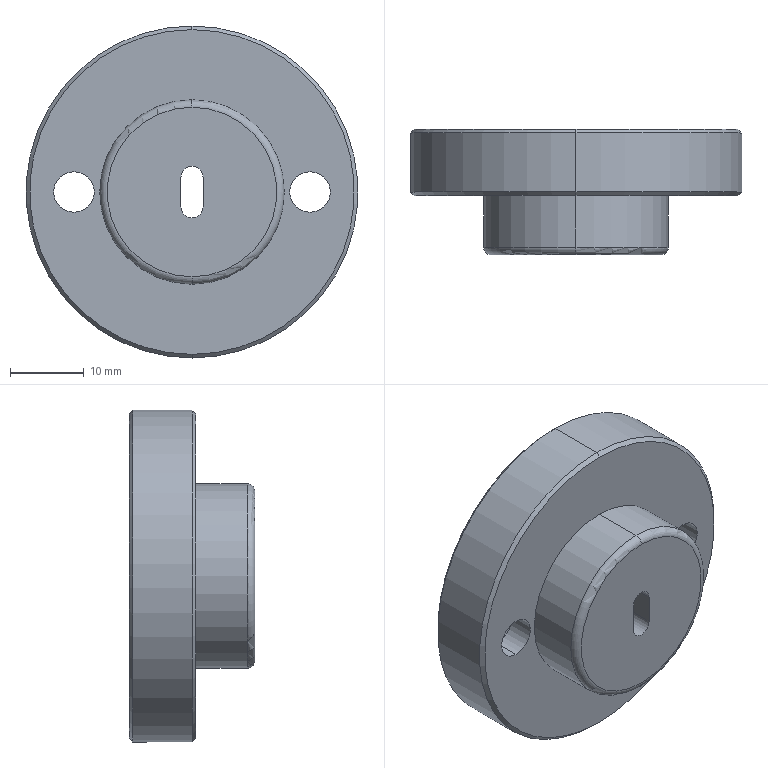Component | SolidWorks | 300-03-1 | 1 solid | 89 faces | box 45 x 17 x 45 mm | volume 16273 mm3 | plane 34 | spline 30 | cylinder 17 | torus 4 | cone 4 | commonest cylinder face diameters 10 x4 5.5 x4 3 x3 10.65 x2 25 x2 45 x2 | material Cr12MoV